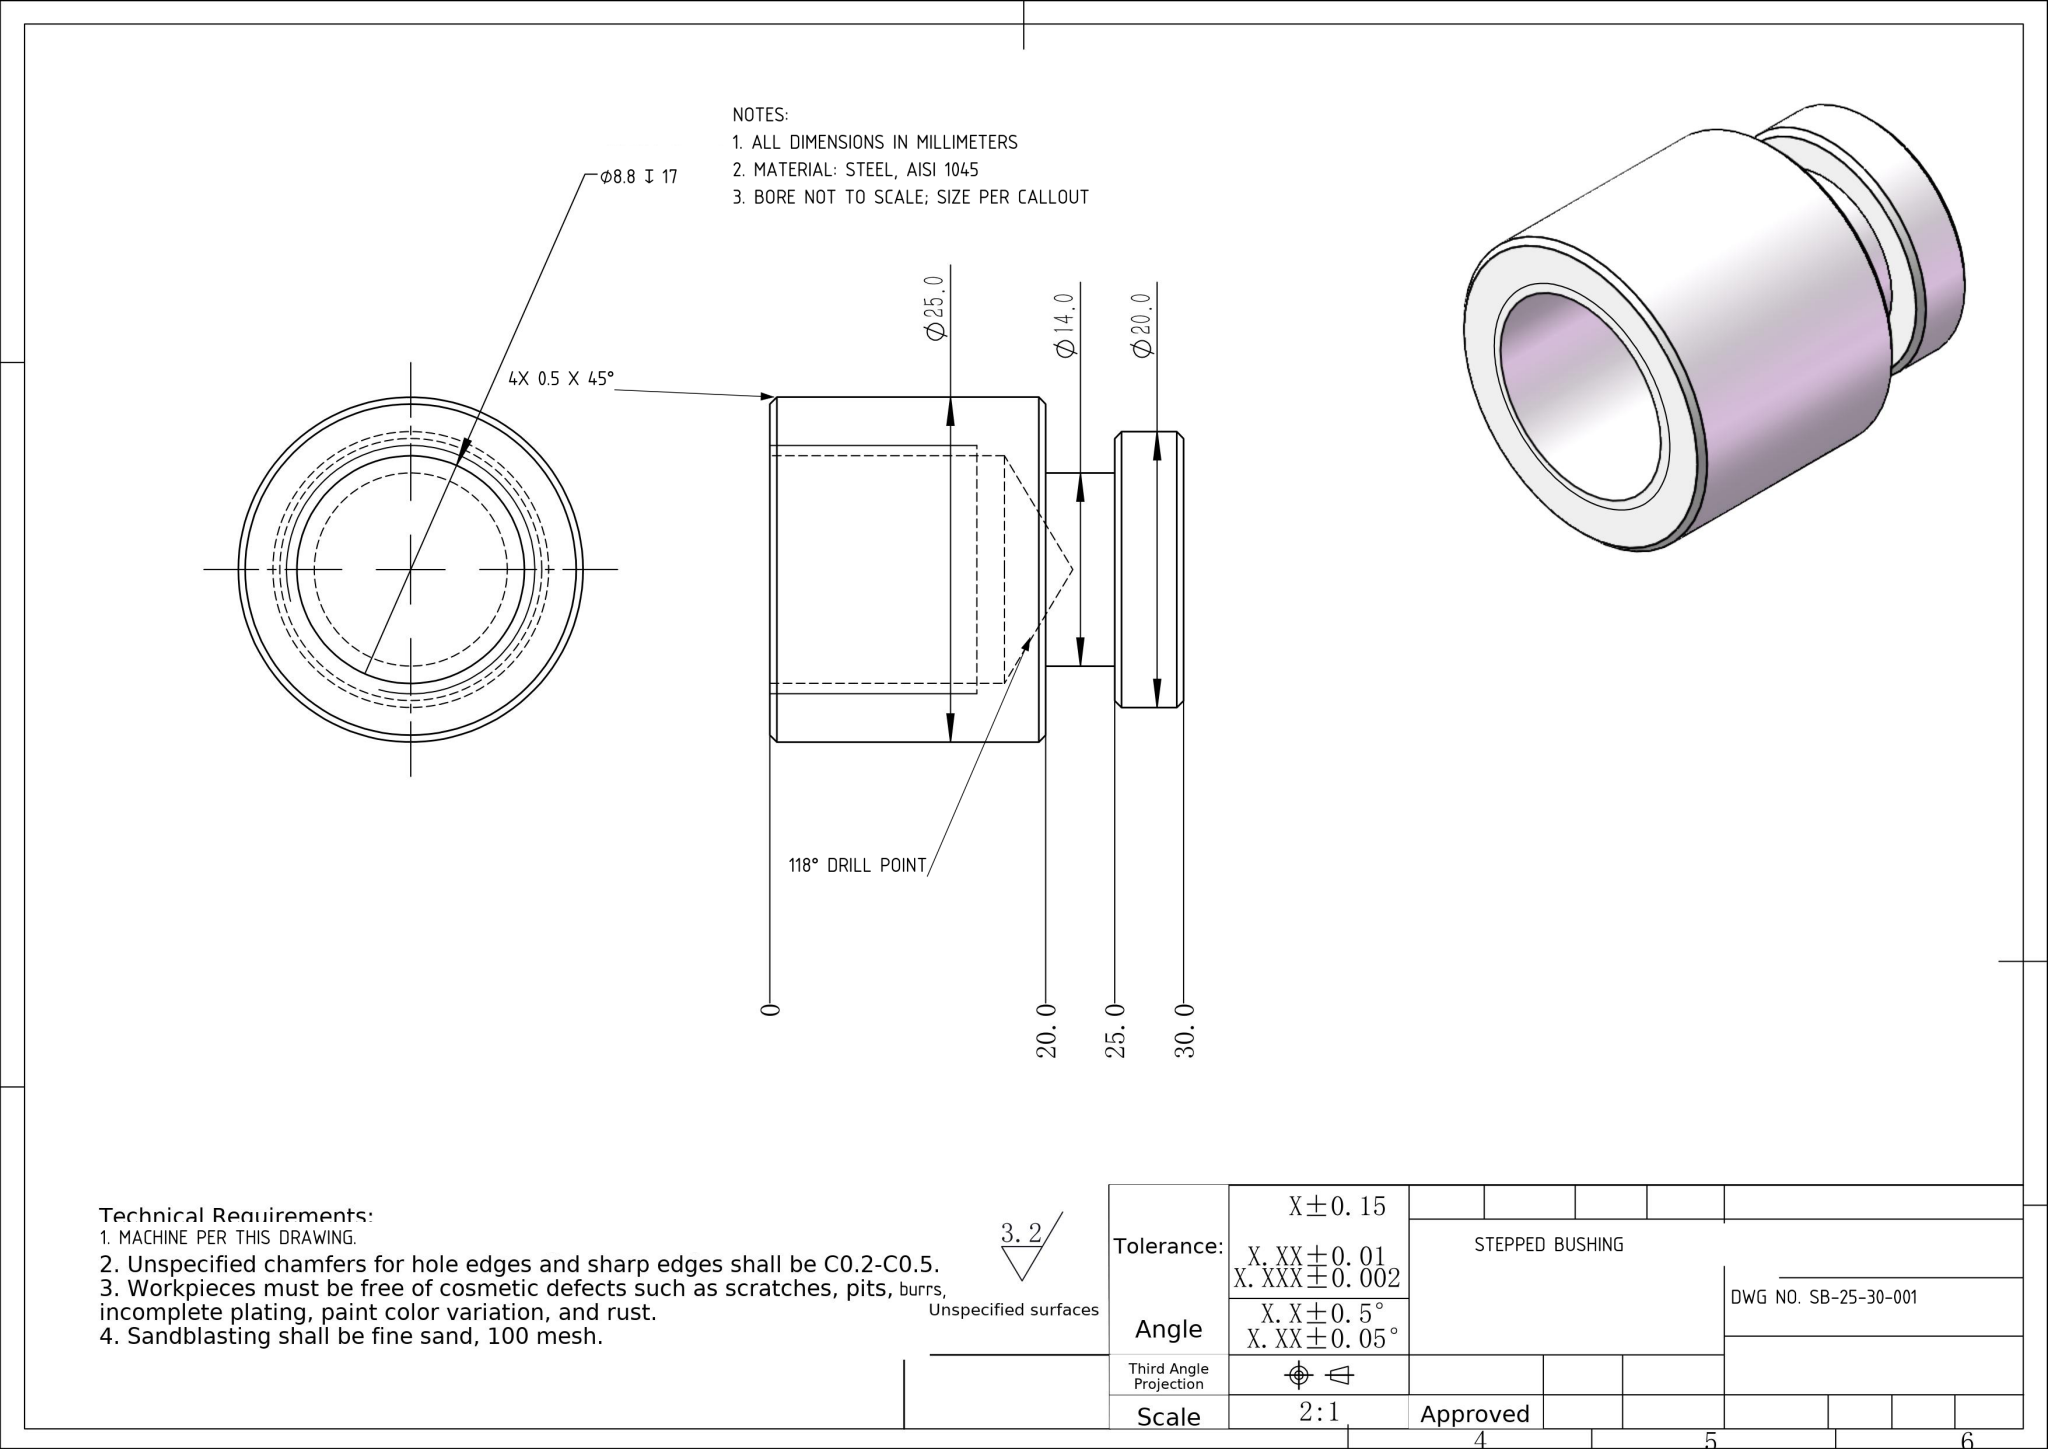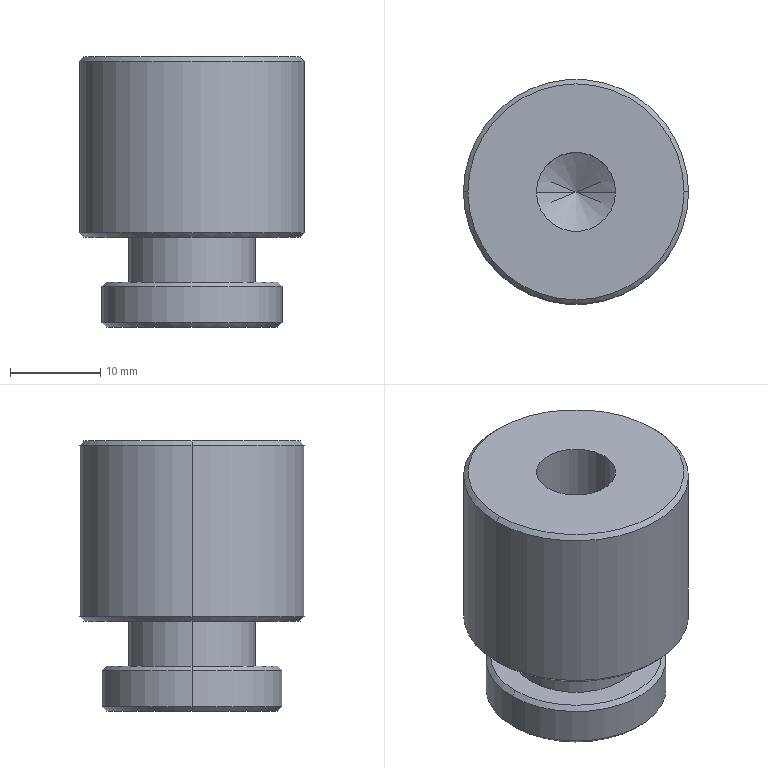Part | NX | mm | 1 solid | 22 faces | box 25 x 25 x 30 mm | volume 11036 mm3 | cone 10 | cylinder 8 | plane 4 | commonest cylinder face diameters 20 x2 8.8 x2 25 x2 14 x2
STEP:
#1=CARTESIAN_POINT('',(109.578,-259.589,0.));
#2=VERTEX_POINT('',#1);
#3=CARTESIAN_POINT('',(128.578,-259.589,0.));
#4=VERTEX_POINT('',#3);
#5=CARTESIAN_POINT('',(119.078,-259.589,0.));
#6=DIRECTION('',(0.,0.,-1.));
#7=DIRECTION('',(1.,0.,0.));
#8=AXIS2_PLACEMENT_3D('',#5,#6,#7);
#9=CIRCLE('',#8,9.5);
#10=EDGE_CURVE('',#2,#4,#9,.T.);
#11=ORIENTED_EDGE('',*,*,#10,.F.);
#12=CARTESIAN_POINT('',(109.078,-259.589,0.5));
#13=VERTEX_POINT('',#12);
#14=CARTESIAN_POINT('',(109.578,-259.589,0.));
#15=DIRECTION('',(-0.7071,0.,0.7071));
#16=VECTOR('',#15,1000.);
#17=LINE('',#14,#16);
#18=EDGE_CURVE('',#2,#13,#17,.T.);
#19=ORIENTED_EDGE('',*,*,#18,.T.);
#20=CARTESIAN_POINT('',(129.078,-259.589,0.5));
#21=VERTEX_POINT('',#20);
#22=CARTESIAN_POINT('',(119.078,-259.589,0.5));
#23=DIRECTION('',(0.,0.,1.));
#24=DIRECTION('',(1.,0.,0.));
#25=AXIS2_PLACEMENT_3D('',#22,#23,#24);
#26=CIRCLE('',#25,10.);
#27=EDGE_CURVE('',#21,#13,#26,.T.);
#28=ORIENTED_EDGE('',*,*,#27,.F.);
#29=CARTESIAN_POINT('',(128.578,-259.589,0.));
#30=DIRECTION('',(0.7071,0.,0.7071));
#31=VECTOR('',#30,1000.);
#32=LINE('',#29,#31);
#33=EDGE_CURVE('',#4,#21,#32,.T.);
#34=ORIENTED_EDGE('',*,*,#33,.F.);
#35=EDGE_LOOP('',(#11,#19,#28,#34));
#36=FACE_OUTER_BOUND('',#35,.T.);
#37=CARTESIAN_POINT('',(119.078,-259.589,0.));
#38=DIRECTION('',(0.,0.,1.));
#39=DIRECTION('',(1.,0.,0.));
#40=AXIS2_PLACEMENT_3D('',#37,#38,#39);
#41=CONICAL_SURFACE('',#40,9.5,0.7854);
#42=ADVANCED_FACE('',(#36),#41,.T.);
#43=CARTESIAN_POINT('',(128.578,-259.589,5.));
#44=VERTEX_POINT('',#43);
#45=CARTESIAN_POINT('',(109.578,-259.589,5.));
#46=VERTEX_POINT('',#45);
#47=CARTESIAN_POINT('',(119.078,-259.589,5.));
#48=DIRECTION('',(0.,0.,1.));
#49=DIRECTION('',(1.,0.,0.));
#50=AXIS2_PLACEMENT_3D('',#47,#48,#49);
#51=CIRCLE('',#50,9.5);
#52=EDGE_CURVE('',#44,#46,#51,.T.);
#53=ORIENTED_EDGE('',*,*,#52,.F.);
#54=CARTESIAN_POINT('',(129.078,-259.589,4.5));
#55=VERTEX_POINT('',#54);
#56=CARTESIAN_POINT('',(128.578,-259.589,5.));
#57=DIRECTION('',(0.7071,0.,-0.7071));
#58=VECTOR('',#57,1000.);
#59=LINE('',#56,#58);
#60=EDGE_CURVE('',#44,#55,#59,.T.);
#61=ORIENTED_EDGE('',*,*,#60,.T.);
#62=CARTESIAN_POINT('',(109.078,-259.589,4.5));
#63=VERTEX_POINT('',#62);
#64=CARTESIAN_POINT('',(119.078,-259.589,4.5));
#65=DIRECTION('',(0.,0.,-1.));
#66=DIRECTION('',(1.,0.,0.));
#67=AXIS2_PLACEMENT_3D('',#64,#65,#66);
#68=CIRCLE('',#67,10.);
#69=EDGE_CURVE('',#63,#55,#68,.T.);
#70=ORIENTED_EDGE('',*,*,#69,.F.);
#71=CARTESIAN_POINT('',(109.578,-259.589,5.));
#72=DIRECTION('',(-0.7071,0.,-0.7071));
#73=VECTOR('',#72,1000.);
#74=LINE('',#71,#73);
#75=EDGE_CURVE('',#46,#63,#74,.T.);
#76=ORIENTED_EDGE('',*,*,#75,.F.);
#77=EDGE_LOOP('',(#53,#61,#70,#76));
#78=FACE_OUTER_BOUND('',#77,.T.);
#79=CARTESIAN_POINT('',(119.078,-259.589,5.));
#80=DIRECTION('',(0.,0.,-1.));
#81=DIRECTION('',(-1.,0.,0.));
#82=AXIS2_PLACEMENT_3D('',#79,#80,#81);
#83=CONICAL_SURFACE('',#82,9.5,0.7854);
#84=ADVANCED_FACE('',(#78),#83,.T.);
#85=ORIENTED_EDGE('',*,*,#69,.T.);
#86=CARTESIAN_POINT('',(129.078,-259.589,10.));
#87=DIRECTION('',(0.,0.,-1.));
#88=VECTOR('',#87,1000.);
#89=LINE('',#86,#88);
#90=EDGE_CURVE('',#55,#21,#89,.T.);
#91=ORIENTED_EDGE('',*,*,#90,.T.);
#92=ORIENTED_EDGE('',*,*,#27,.T.);
#93=CARTESIAN_POINT('',(109.078,-259.589,10.));
#94=DIRECTION('',(0.,0.,-1.));
#95=VECTOR('',#94,1000.);
#96=LINE('',#93,#95);
#97=EDGE_CURVE('',#63,#13,#96,.T.);
#98=ORIENTED_EDGE('',*,*,#97,.F.);
#99=EDGE_LOOP('',(#85,#91,#92,#98));
#100=FACE_OUTER_BOUND('',#99,.T.);
#101=CARTESIAN_POINT('',(119.078,-259.589,10.));
#102=DIRECTION('',(0.,0.,-1.));
#103=DIRECTION('',(-1.,0.,0.));
#104=AXIS2_PLACEMENT_3D('',#101,#102,#103);
#105=CYLINDRICAL_SURFACE('',#104,10.);
#106=ADVANCED_FACE('',(#100),#105,.T.);
#107=CARTESIAN_POINT('',(114.678,-259.589,13.));
#108=VERTEX_POINT('',#107);
#109=CARTESIAN_POINT('',(123.478,-259.589,13.));
#110=VERTEX_POINT('',#109);
#111=CARTESIAN_POINT('',(119.078,-259.589,13.));
#112=DIRECTION('',(0.,0.,1.));
#113=DIRECTION('',(1.,0.,0.));
#114=AXIS2_PLACEMENT_3D('',#111,#112,#113);
#115=CIRCLE('',#114,4.4);
#116=EDGE_CURVE('',#108,#110,#115,.T.);
#117=ORIENTED_EDGE('',*,*,#116,.F.);
#118=CARTESIAN_POINT('',(114.678,-259.589,30.));
#119=VERTEX_POINT('',#118);
#120=CARTESIAN_POINT('',(114.678,-259.589,30.));
#121=DIRECTION('',(0.,0.,1.));
#122=VECTOR('',#121,1000.);
#123=LINE('',#120,#122);
#124=EDGE_CURVE('',#108,#119,#123,.T.);
#125=ORIENTED_EDGE('',*,*,#124,.T.);
#126=CARTESIAN_POINT('',(123.478,-259.589,30.));
#127=VERTEX_POINT('',#126);
#128=CARTESIAN_POINT('',(119.078,-259.589,30.));
#129=DIRECTION('',(0.,0.,1.));
#130=DIRECTION('',(1.,0.,0.));
#131=AXIS2_PLACEMENT_3D('',#128,#129,#130);
#132=CIRCLE('',#131,4.4);
#133=EDGE_CURVE('',#119,#127,#132,.T.);
#134=ORIENTED_EDGE('',*,*,#133,.T.);
#135=CARTESIAN_POINT('',(123.478,-259.589,30.));
#136=DIRECTION('',(0.,0.,1.));
#137=VECTOR('',#136,1000.);
#138=LINE('',#135,#137);
#139=EDGE_CURVE('',#110,#127,#138,.T.);
#140=ORIENTED_EDGE('',*,*,#139,.F.);
#141=EDGE_LOOP('',(#117,#125,#134,#140));
#142=FACE_OUTER_BOUND('',#141,.T.);
#143=CARTESIAN_POINT('',(119.078,-259.589,30.));
#144=DIRECTION('',(0.,0.,1.));
#145=DIRECTION('',(1.,0.,0.));
#146=AXIS2_PLACEMENT_3D('',#143,#144,#145);
#147=CYLINDRICAL_SURFACE('',#146,4.4);
#148=ADVANCED_FACE('',(#142),#147,.F.);
#149=CARTESIAN_POINT('',(119.078,-259.589,10.356));
#150=VERTEX_POINT('',#149);
#151=CARTESIAN_POINT('',(123.478,-259.589,13.));
#152=DIRECTION('',(0.8572,0.,0.515));
#153=VECTOR('',#152,1000.);
#154=LINE('',#151,#153);
#155=EDGE_CURVE('',#150,#110,#154,.T.);
#156=ORIENTED_EDGE('',*,*,#155,.F.);
#157=CARTESIAN_POINT('',(114.678,-259.589,13.));
#158=DIRECTION('',(-0.8572,0.,0.515));
#159=VECTOR('',#158,1000.);
#160=LINE('',#157,#159);
#161=EDGE_CURVE('',#150,#108,#160,.T.);
#162=ORIENTED_EDGE('',*,*,#161,.T.);
#163=ORIENTED_EDGE('',*,*,#116,.T.);
#164=EDGE_LOOP('',(#156,#162,#163));
#165=FACE_OUTER_BOUND('',#164,.T.);
#166=CARTESIAN_POINT('',(119.078,-259.589,13.));
#167=DIRECTION('',(0.,0.,1.));
#168=DIRECTION('',(1.,0.,0.));
#169=AXIS2_PLACEMENT_3D('',#166,#167,#168);
#170=CONICAL_SURFACE('',#169,4.4,1.03);
#171=ADVANCED_FACE('',(#165),#170,.F.);
#172=CARTESIAN_POINT('',(107.078,-259.589,10.));
#173=VERTEX_POINT('',#172);
#174=CARTESIAN_POINT('',(131.078,-259.589,10.));
#175=VERTEX_POINT('',#174);
#176=CARTESIAN_POINT('',(119.078,-259.589,10.));
#177=DIRECTION('',(0.,0.,-1.));
#178=DIRECTION('',(1.,0.,0.));
#179=AXIS2_PLACEMENT_3D('',#176,#177,#178);
#180=CIRCLE('',#179,12.);
#181=EDGE_CURVE('',#173,#175,#180,.T.);
#182=ORIENTED_EDGE('',*,*,#181,.F.);
#183=CARTESIAN_POINT('',(106.578,-259.589,10.5));
#184=VERTEX_POINT('',#183);
#185=CARTESIAN_POINT('',(106.578,-259.589,10.5));
#186=DIRECTION('',(-0.7071,0.,0.7071));
#187=VECTOR('',#186,1000.);
#188=LINE('',#185,#187);
#189=EDGE_CURVE('',#173,#184,#188,.T.);
#190=ORIENTED_EDGE('',*,*,#189,.T.);
#191=CARTESIAN_POINT('',(131.578,-259.589,10.5));
#192=VERTEX_POINT('',#191);
#193=CARTESIAN_POINT('',(119.078,-259.589,10.5));
#194=DIRECTION('',(0.,0.,1.));
#195=DIRECTION('',(1.,0.,0.));
#196=AXIS2_PLACEMENT_3D('',#193,#194,#195);
#197=CIRCLE('',#196,12.5);
#198=EDGE_CURVE('',#192,#184,#197,.T.);
#199=ORIENTED_EDGE('',*,*,#198,.F.);
#200=CARTESIAN_POINT('',(131.578,-259.589,10.5));
#201=DIRECTION('',(0.7071,0.,0.7071));
#202=VECTOR('',#201,1000.);
#203=LINE('',#200,#202);
#204=EDGE_CURVE('',#175,#192,#203,.T.);
#205=ORIENTED_EDGE('',*,*,#204,.F.);
#206=EDGE_LOOP('',(#182,#190,#199,#205));
#207=FACE_OUTER_BOUND('',#206,.T.);
#208=CARTESIAN_POINT('',(119.078,-259.589,10.5));
#209=DIRECTION('',(0.,0.,1.));
#210=DIRECTION('',(1.,0.,0.));
#211=AXIS2_PLACEMENT_3D('',#208,#209,#210);
#212=CONICAL_SURFACE('',#211,12.5,0.7854);
#213=ADVANCED_FACE('',(#207),#212,.T.);
#214=CARTESIAN_POINT('',(131.078,-259.589,30.));
#215=VERTEX_POINT('',#214);
#216=CARTESIAN_POINT('',(107.078,-259.589,30.));
#217=VERTEX_POINT('',#216);
#218=CARTESIAN_POINT('',(119.078,-259.589,30.));
#219=DIRECTION('',(0.,0.,1.));
#220=DIRECTION('',(1.,0.,0.));
#221=AXIS2_PLACEMENT_3D('',#218,#219,#220);
#222=CIRCLE('',#221,12.);
#223=EDGE_CURVE('',#215,#217,#222,.T.);
#224=ORIENTED_EDGE('',*,*,#223,.F.);
#225=CARTESIAN_POINT('',(131.578,-259.589,29.5));
#226=VERTEX_POINT('',#225);
#227=CARTESIAN_POINT('',(131.078,-259.589,30.));
#228=DIRECTION('',(0.7071,0.,-0.7071));
#229=VECTOR('',#228,1000.);
#230=LINE('',#227,#229);
#231=EDGE_CURVE('',#215,#226,#230,.T.);
#232=ORIENTED_EDGE('',*,*,#231,.T.);
#233=CARTESIAN_POINT('',(106.578,-259.589,29.5));
#234=VERTEX_POINT('',#233);
#235=CARTESIAN_POINT('',(119.078,-259.589,29.5));
#236=DIRECTION('',(0.,0.,-1.));
#237=DIRECTION('',(1.,0.,0.));
#238=AXIS2_PLACEMENT_3D('',#235,#236,#237);
#239=CIRCLE('',#238,12.5);
#240=EDGE_CURVE('',#234,#226,#239,.T.);
#241=ORIENTED_EDGE('',*,*,#240,.F.);
#242=CARTESIAN_POINT('',(107.078,-259.589,30.));
#243=DIRECTION('',(-0.7071,0.,-0.7071));
#244=VECTOR('',#243,1000.);
#245=LINE('',#242,#244);
#246=EDGE_CURVE('',#217,#234,#245,.T.);
#247=ORIENTED_EDGE('',*,*,#246,.F.);
#248=EDGE_LOOP('',(#224,#232,#241,#247));
#249=FACE_OUTER_BOUND('',#248,.T.);
#250=CARTESIAN_POINT('',(119.078,-259.589,30.));
#251=DIRECTION('',(0.,0.,-1.));
#252=DIRECTION('',(-1.,0.,0.));
#253=AXIS2_PLACEMENT_3D('',#250,#251,#252);
#254=CONICAL_SURFACE('',#253,12.,0.7854);
#255=ADVANCED_FACE('',(#249),#254,.T.);
#256=ORIENTED_EDGE('',*,*,#240,.T.);
#257=CARTESIAN_POINT('',(131.578,-259.589,25.));
#258=DIRECTION('',(0.,0.,-1.));
#259=VECTOR('',#258,1000.);
#260=LINE('',#257,#259);
#261=EDGE_CURVE('',#226,#192,#260,.T.);
#262=ORIENTED_EDGE('',*,*,#261,.T.);
#263=ORIENTED_EDGE('',*,*,#198,.T.);
#264=CARTESIAN_POINT('',(106.578,-259.589,25.));
#265=DIRECTION('',(0.,0.,-1.));
#266=VECTOR('',#265,1000.);
#267=LINE('',#264,#266);
#268=EDGE_CURVE('',#234,#184,#267,.T.);
#269=ORIENTED_EDGE('',*,*,#268,.F.);
#270=EDGE_LOOP('',(#256,#262,#263,#269));
#271=FACE_OUTER_BOUND('',#270,.T.);
#272=CARTESIAN_POINT('',(119.078,-259.589,25.));
#273=DIRECTION('',(0.,0.,-1.));
#274=DIRECTION('',(-1.,0.,0.));
#275=AXIS2_PLACEMENT_3D('',#272,#273,#274);
#276=CYLINDRICAL_SURFACE('',#275,12.5);
#277=ADVANCED_FACE('',(#271),#276,.T.);
#278=CARTESIAN_POINT('',(126.078,-259.589,5.));
#279=VERTEX_POINT('',#278);
#280=CARTESIAN_POINT('',(112.078,-259.589,5.));
#281=VERTEX_POINT('',#280);
#282=CARTESIAN_POINT('',(119.078,-259.589,5.));
#283=DIRECTION('',(0.,0.,1.));
#284=DIRECTION('',(1.,0.,0.));
#285=AXIS2_PLACEMENT_3D('',#282,#283,#284);
#286=CIRCLE('',#285,7.);
#287=EDGE_CURVE('',#279,#281,#286,.T.);
#288=ORIENTED_EDGE('',*,*,#287,.T.);
#289=CARTESIAN_POINT('',(112.078,-259.589,10.));
#290=VERTEX_POINT('',#289);
#291=CARTESIAN_POINT('',(112.078,-259.589,5.));
#292=DIRECTION('',(0.,0.,1.));
#293=VECTOR('',#292,1000.);
#294=LINE('',#291,#293);
#295=EDGE_CURVE('',#281,#290,#294,.T.);
#296=ORIENTED_EDGE('',*,*,#295,.T.);
#297=CARTESIAN_POINT('',(126.078,-259.589,10.));
#298=VERTEX_POINT('',#297);
#299=CARTESIAN_POINT('',(119.078,-259.589,10.));
#300=DIRECTION('',(0.,0.,1.));
#301=DIRECTION('',(1.,0.,0.));
#302=AXIS2_PLACEMENT_3D('',#299,#300,#301);
#303=CIRCLE('',#302,7.);
#304=EDGE_CURVE('',#298,#290,#303,.T.);
#305=ORIENTED_EDGE('',*,*,#304,.F.);
#306=CARTESIAN_POINT('',(126.078,-259.589,5.));
#307=DIRECTION('',(0.,0.,1.));
#308=VECTOR('',#307,1000.);
#309=LINE('',#306,#308);
#310=EDGE_CURVE('',#279,#298,#309,.T.);
#311=ORIENTED_EDGE('',*,*,#310,.F.);
#312=EDGE_LOOP('',(#288,#296,#305,#311));
#313=FACE_OUTER_BOUND('',#312,.T.);
#314=CARTESIAN_POINT('',(119.078,-259.589,5.));
#315=DIRECTION('',(0.,0.,1.));
#316=DIRECTION('',(1.,0.,0.));
#317=AXIS2_PLACEMENT_3D('',#314,#315,#316);
#318=CYLINDRICAL_SURFACE('',#317,7.);
#319=ADVANCED_FACE('',(#313),#318,.T.);
#320=CARTESIAN_POINT('',(119.078,-259.589,5.));
#321=DIRECTION('',(0.,0.,1.));
#322=DIRECTION('',(1.,0.,0.));
#323=AXIS2_PLACEMENT_3D('',#320,#321,#322);
#324=CIRCLE('',#323,9.5);
#325=EDGE_CURVE('',#46,#44,#324,.T.);
#326=ORIENTED_EDGE('',*,*,#325,.T.);
#327=ORIENTED_EDGE('',*,*,#52,.T.);
#328=EDGE_LOOP('',(#326,#327));
#329=FACE_OUTER_BOUND('',#328,.T.);
#330=ORIENTED_EDGE('',*,*,#287,.F.);
#331=CARTESIAN_POINT('',(119.078,-259.589,5.));
#332=DIRECTION('',(0.,0.,1.));
#333=DIRECTION('',(1.,0.,0.));
#334=AXIS2_PLACEMENT_3D('',#331,#332,#333);
#335=CIRCLE('',#334,7.);
#336=EDGE_CURVE('',#281,#279,#335,.T.);
#337=ORIENTED_EDGE('',*,*,#336,.F.);
#338=EDGE_LOOP('',(#330,#337));
#339=FACE_BOUND('',#338,.T.);
#340=CARTESIAN_POINT('',(119.078,-259.589,5.));
#341=DIRECTION('',(0.,0.,1.));
#342=DIRECTION('',(1.,0.,0.));
#343=AXIS2_PLACEMENT_3D('',#340,#341,#342);
#344=PLANE('',#343);
#345=ADVANCED_FACE('',(#329,#339),#344,.T.);
#346=CARTESIAN_POINT('',(119.078,-259.589,10.));
#347=DIRECTION('',(0.,0.,-1.));
#348=DIRECTION('',(1.,0.,0.));
#349=AXIS2_PLACEMENT_3D('',#346,#347,#348);
#350=CIRCLE('',#349,12.);
#351=EDGE_CURVE('',#175,#173,#350,.T.);
#352=ORIENTED_EDGE('',*,*,#351,.T.);
#353=ORIENTED_EDGE('',*,*,#181,.T.);
#354=EDGE_LOOP('',(#352,#353));
#355=FACE_OUTER_BOUND('',#354,.T.);
#356=ORIENTED_EDGE('',*,*,#304,.T.);
#357=CARTESIAN_POINT('',(119.078,-259.589,10.));
#358=DIRECTION('',(0.,0.,1.));
#359=DIRECTION('',(1.,0.,0.));
#360=AXIS2_PLACEMENT_3D('',#357,#358,#359);
#361=CIRCLE('',#360,7.);
#362=EDGE_CURVE('',#290,#298,#361,.T.);
#363=ORIENTED_EDGE('',*,*,#362,.T.);
#364=EDGE_LOOP('',(#356,#363));
#365=FACE_BOUND('',#364,.T.);
#366=CARTESIAN_POINT('',(119.078,-259.589,10.));
#367=DIRECTION('',(0.,0.,1.));
#368=DIRECTION('',(1.,0.,0.));
#369=AXIS2_PLACEMENT_3D('',#366,#367,#368);
#370=PLANE('',#369);
#371=ADVANCED_FACE('',(#355,#365),#370,.F.);
#372=ORIENTED_EDGE('',*,*,#295,.F.);
#373=ORIENTED_EDGE('',*,*,#336,.T.);
#374=ORIENTED_EDGE('',*,*,#310,.T.);
#375=ORIENTED_EDGE('',*,*,#362,.F.);
#376=EDGE_LOOP('',(#372,#373,#374,#375));
#377=FACE_OUTER_BOUND('',#376,.T.);
#378=CARTESIAN_POINT('',(119.078,-259.589,5.));
#379=DIRECTION('',(0.,0.,1.));
#380=DIRECTION('',(1.,0.,0.));
#381=AXIS2_PLACEMENT_3D('',#378,#379,#380);
#382=CYLINDRICAL_SURFACE('',#381,7.);
#383=ADVANCED_FACE('',(#377),#382,.T.);
#384=CARTESIAN_POINT('',(119.078,-259.589,30.));
#385=DIRECTION('',(0.,0.,1.));
#386=DIRECTION('',(1.,0.,0.));
#387=AXIS2_PLACEMENT_3D('',#384,#385,#386);
#388=CIRCLE('',#387,4.4);
#389=EDGE_CURVE('',#127,#119,#388,.T.);
#390=ORIENTED_EDGE('',*,*,#389,.F.);
#391=ORIENTED_EDGE('',*,*,#133,.F.);
#392=EDGE_LOOP('',(#390,#391));
#393=FACE_BOUND('',#392,.T.);
#394=CARTESIAN_POINT('',(119.078,-259.589,30.));
#395=DIRECTION('',(0.,0.,1.));
#396=DIRECTION('',(1.,0.,0.));
#397=AXIS2_PLACEMENT_3D('',#394,#395,#396);
#398=CIRCLE('',#397,12.);
#399=EDGE_CURVE('',#217,#215,#398,.T.);
#400=ORIENTED_EDGE('',*,*,#399,.T.);
#401=ORIENTED_EDGE('',*,*,#223,.T.);
#402=EDGE_LOOP('',(#400,#401));
#403=FACE_OUTER_BOUND('',#402,.T.);
#404=CARTESIAN_POINT('',(119.078,-259.589,30.));
#405=DIRECTION('',(0.,0.,1.));
#406=DIRECTION('',(1.,0.,0.));
#407=AXIS2_PLACEMENT_3D('',#404,#405,#406);
#408=PLANE('',#407);
#409=ADVANCED_FACE('',(#393,#403),#408,.T.);
#410=ORIENTED_EDGE('',*,*,#261,.F.);
#411=CARTESIAN_POINT('',(119.078,-259.589,29.5));
#412=DIRECTION('',(0.,0.,-1.));
#413=DIRECTION('',(1.,0.,0.));
#414=AXIS2_PLACEMENT_3D('',#411,#412,#413);
#415=CIRCLE('',#414,12.5);
#416=EDGE_CURVE('',#226,#234,#415,.T.);
#417=ORIENTED_EDGE('',*,*,#416,.T.);
#418=ORIENTED_EDGE('',*,*,#268,.T.);
#419=CARTESIAN_POINT('',(119.078,-259.589,10.5));
#420=DIRECTION('',(0.,0.,1.));
#421=DIRECTION('',(1.,0.,0.));
#422=AXIS2_PLACEMENT_3D('',#419,#420,#421);
#423=CIRCLE('',#422,12.5);
#424=EDGE_CURVE('',#184,#192,#423,.T.);
#425=ORIENTED_EDGE('',*,*,#424,.T.);
#426=EDGE_LOOP('',(#410,#417,#418,#425));
#427=FACE_OUTER_BOUND('',#426,.T.);
#428=CARTESIAN_POINT('',(119.078,-259.589,25.));
#429=DIRECTION('',(0.,0.,-1.));
#430=DIRECTION('',(-1.,0.,0.));
#431=AXIS2_PLACEMENT_3D('',#428,#429,#430);
#432=CYLINDRICAL_SURFACE('',#431,12.5);
#433=ADVANCED_FACE('',(#427),#432,.T.);
#434=ORIENTED_EDGE('',*,*,#231,.F.);
#435=ORIENTED_EDGE('',*,*,#399,.F.);
#436=ORIENTED_EDGE('',*,*,#246,.T.);
#437=ORIENTED_EDGE('',*,*,#416,.F.);
#438=EDGE_LOOP('',(#434,#435,#436,#437));
#439=FACE_OUTER_BOUND('',#438,.T.);
#440=CARTESIAN_POINT('',(119.078,-259.589,30.));
#441=DIRECTION('',(0.,0.,-1.));
#442=DIRECTION('',(-1.,0.,0.));
#443=AXIS2_PLACEMENT_3D('',#440,#441,#442);
#444=CONICAL_SURFACE('',#443,12.,0.7854);
#445=ADVANCED_FACE('',(#439),#444,.T.);
#446=ORIENTED_EDGE('',*,*,#189,.F.);
#447=ORIENTED_EDGE('',*,*,#351,.F.);
#448=ORIENTED_EDGE('',*,*,#204,.T.);
#449=ORIENTED_EDGE('',*,*,#424,.F.);
#450=EDGE_LOOP('',(#446,#447,#448,#449));
#451=FACE_OUTER_BOUND('',#450,.T.);
#452=CARTESIAN_POINT('',(119.078,-259.589,10.5));
#453=DIRECTION('',(0.,0.,1.));
#454=DIRECTION('',(1.,0.,0.));
#455=AXIS2_PLACEMENT_3D('',#452,#453,#454);
#456=CONICAL_SURFACE('',#455,12.5,0.7854);
#457=ADVANCED_FACE('',(#451),#456,.T.);
#458=ORIENTED_EDGE('',*,*,#161,.F.);
#459=ORIENTED_EDGE('',*,*,#155,.T.);
#460=CARTESIAN_POINT('',(119.078,-259.589,13.));
#461=DIRECTION('',(0.,0.,1.));
#462=DIRECTION('',(1.,0.,0.));
#463=AXIS2_PLACEMENT_3D('',#460,#461,#462);
#464=CIRCLE('',#463,4.4);
#465=EDGE_CURVE('',#110,#108,#464,.T.);
#466=ORIENTED_EDGE('',*,*,#465,.T.);
#467=EDGE_LOOP('',(#458,#459,#466));
#468=FACE_OUTER_BOUND('',#467,.T.);
#469=CARTESIAN_POINT('',(119.078,-259.589,13.));
#470=DIRECTION('',(0.,0.,1.));
#471=DIRECTION('',(1.,0.,0.));
#472=AXIS2_PLACEMENT_3D('',#469,#470,#471);
#473=CONICAL_SURFACE('',#472,4.4,1.03);
#474=ADVANCED_FACE('',(#468),#473,.F.);
#475=ORIENTED_EDGE('',*,*,#124,.F.);
#476=ORIENTED_EDGE('',*,*,#465,.F.);
#477=ORIENTED_EDGE('',*,*,#139,.T.);
#478=ORIENTED_EDGE('',*,*,#389,.T.);
#479=EDGE_LOOP('',(#475,#476,#477,#478));
#480=FACE_OUTER_BOUND('',#479,.T.);
#481=CARTESIAN_POINT('',(119.078,-259.589,30.));
#482=DIRECTION('',(0.,0.,1.));
#483=DIRECTION('',(1.,0.,0.));
#484=AXIS2_PLACEMENT_3D('',#481,#482,#483);
#485=CYLINDRICAL_SURFACE('',#484,4.4);
#486=ADVANCED_FACE('',(#480),#485,.F.);
#487=ORIENTED_EDGE('',*,*,#90,.F.);
#488=CARTESIAN_POINT('',(119.078,-259.589,4.5));
#489=DIRECTION('',(0.,0.,-1.));
#490=DIRECTION('',(1.,0.,0.));
#491=AXIS2_PLACEMENT_3D('',#488,#489,#490);
#492=CIRCLE('',#491,10.);
#493=EDGE_CURVE('',#55,#63,#492,.T.);
#494=ORIENTED_EDGE('',*,*,#493,.T.);
#495=ORIENTED_EDGE('',*,*,#97,.T.);
#496=CARTESIAN_POINT('',(119.078,-259.589,0.5));
#497=DIRECTION('',(0.,0.,1.));
#498=DIRECTION('',(1.,0.,0.));
#499=AXIS2_PLACEMENT_3D('',#496,#497,#498);
#500=CIRCLE('',#499,10.);
#501=EDGE_CURVE('',#13,#21,#500,.T.);
#502=ORIENTED_EDGE('',*,*,#501,.T.);
#503=EDGE_LOOP('',(#487,#494,#495,#502));
#504=FACE_OUTER_BOUND('',#503,.T.);
#505=CARTESIAN_POINT('',(119.078,-259.589,10.));
#506=DIRECTION('',(0.,0.,-1.));
#507=DIRECTION('',(-1.,0.,0.));
#508=AXIS2_PLACEMENT_3D('',#505,#506,#507);
#509=CYLINDRICAL_SURFACE('',#508,10.);
#510=ADVANCED_FACE('',(#504),#509,.T.);
#511=CARTESIAN_POINT('',(119.078,-259.589,0.));
#512=DIRECTION('',(0.,0.,-1.));
#513=DIRECTION('',(1.,0.,0.));
#514=AXIS2_PLACEMENT_3D('',#511,#512,#513);
#515=CIRCLE('',#514,9.5);
#516=EDGE_CURVE('',#4,#2,#515,.T.);
#517=ORIENTED_EDGE('',*,*,#516,.T.);
#518=ORIENTED_EDGE('',*,*,#10,.T.);
#519=EDGE_LOOP('',(#517,#518));
#520=FACE_OUTER_BOUND('',#519,.T.);
#521=CARTESIAN_POINT('',(119.078,-259.589,0.));
#522=DIRECTION('',(0.,0.,1.));
#523=DIRECTION('',(1.,0.,0.));
#524=AXIS2_PLACEMENT_3D('',#521,#522,#523);
#525=PLANE('',#524);
#526=ADVANCED_FACE('',(#520),#525,.F.);
#527=ORIENTED_EDGE('',*,*,#60,.F.);
#528=ORIENTED_EDGE('',*,*,#325,.F.);
#529=ORIENTED_EDGE('',*,*,#75,.T.);
#530=ORIENTED_EDGE('',*,*,#493,.F.);
#531=EDGE_LOOP('',(#527,#528,#529,#530));
#532=FACE_OUTER_BOUND('',#531,.T.);
#533=CARTESIAN_POINT('',(119.078,-259.589,5.));
#534=DIRECTION('',(0.,0.,-1.));
#535=DIRECTION('',(-1.,0.,0.));
#536=AXIS2_PLACEMENT_3D('',#533,#534,#535);
#537=CONICAL_SURFACE('',#536,9.5,0.7854);
#538=ADVANCED_FACE('',(#532),#537,.T.);
#539=ORIENTED_EDGE('',*,*,#18,.F.);
#540=ORIENTED_EDGE('',*,*,#516,.F.);
#541=ORIENTED_EDGE('',*,*,#33,.T.);
#542=ORIENTED_EDGE('',*,*,#501,.F.);
#543=EDGE_LOOP('',(#539,#540,#541,#542));
#544=FACE_OUTER_BOUND('',#543,.T.);
#545=CARTESIAN_POINT('',(119.078,-259.589,0.));
#546=DIRECTION('',(0.,0.,1.));
#547=DIRECTION('',(1.,0.,0.));
#548=AXIS2_PLACEMENT_3D('',#545,#546,#547);
#549=CONICAL_SURFACE('',#548,9.5,0.7854);
#550=ADVANCED_FACE('',(#544),#549,.T.);
#551=CLOSED_SHELL('',(#42,#84,#106,#148,#171,#213,#255,#277,#319,#345,#371,#383,#409,#433,#445,#457,#474,#486,#510,#526,#538,#550));
#552=MANIFOLD_SOLID_BREP('',#551);
#553=CARTESIAN_POINT('',(0.,0.,0.));
#554=DIRECTION('',(0.,0.,1.));
#555=DIRECTION('',(1.,0.,0.));
#556=AXIS2_PLACEMENT_3D('',#553,#554,#555);
#557=(LENGTH_UNIT()NAMED_UNIT(*)SI_UNIT(.MILLI.,.METRE.));
#558=UNCERTAINTY_MEASURE_WITH_UNIT(LENGTH_MEASURE(0.00001),#557,'','');
#559=(NAMED_UNIT(*)PLANE_ANGLE_UNIT()SI_UNIT($,.RADIAN.));
#560=(NAMED_UNIT(*)SI_UNIT($,.STERADIAN.)SOLID_ANGLE_UNIT());
#561=(GEOMETRIC_REPRESENTATION_CONTEXT(3)GLOBAL_UNCERTAINTY_ASSIGNED_CONTEXT((#558))GLOBAL_UNIT_ASSIGNED_CONTEXT((#557,#559,#560))REPRESENTATION_CONTEXT('',''));
#562=ADVANCED_BREP_SHAPE_REPRESENTATION('',(#552,#556),#561);